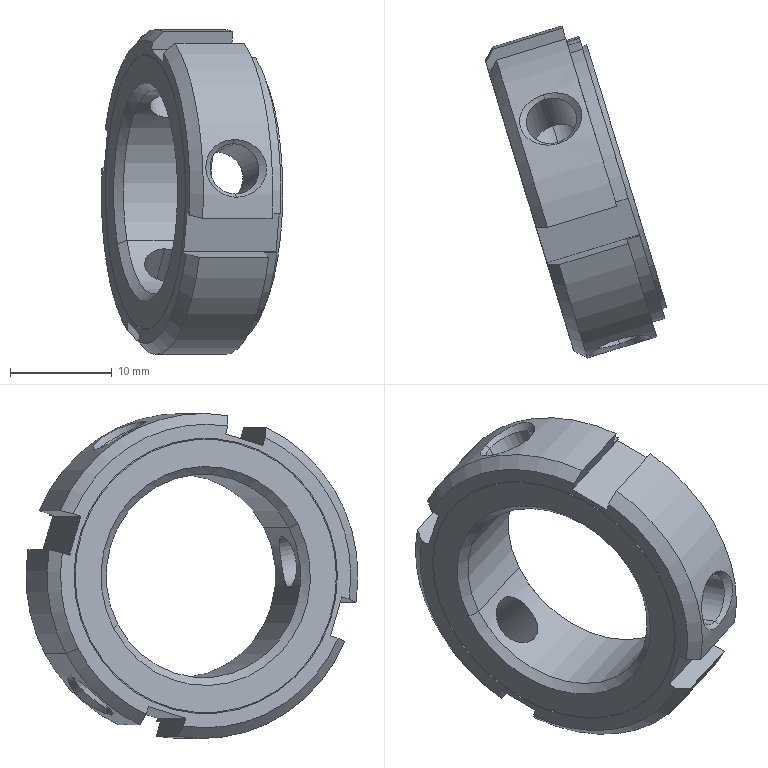Component | SolidWorks | v1ZHXTPLNY20SB1-1_v1ZHXTPLNY20xSB1-1 | 1 solid | 57 faces | box 17.86 x 32.69 x 32 mm | volume 3876 mm3 | cylinder 20 | plane 20 | cone 15 | torus 2 | commonest cylinder face diameters 5.02 x6 29 x5 32 x5 27 x2 20.02 x2